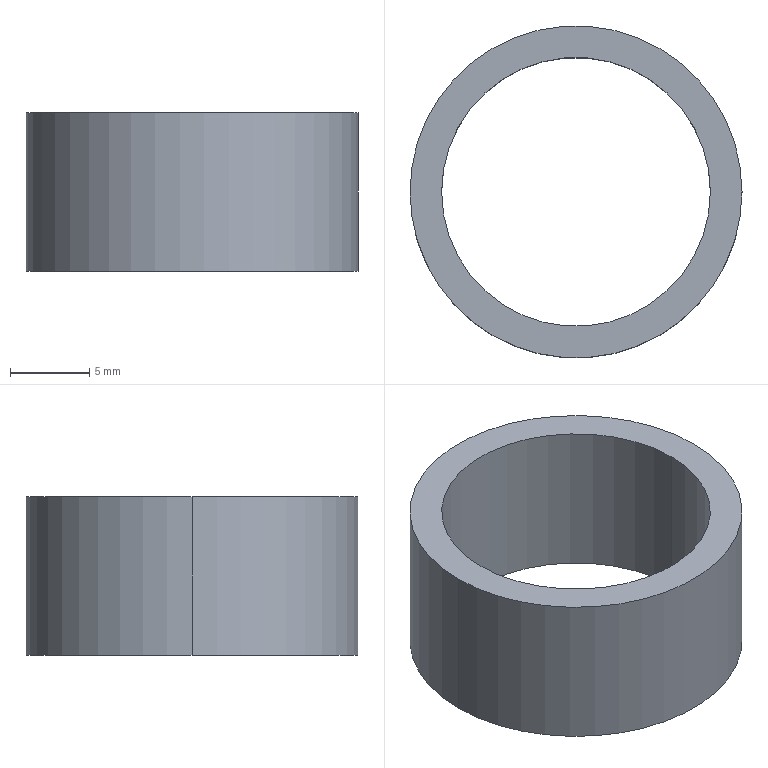Component | SolidWorks | ZDG0406-A03-P07-X1-1 | 1 solid | 6 faces | box 21 x 21 x 10 mm | volume 1194 mm3 | cylinder 4 | plane 2 | commonest cylinder face diameters 17 x2 21 x2 | material 45#
build123d program:
from build123d import *

# Parameters (mm, degrees)
SKETCH1_R           = 10.5
SKETCH1_R_2         = 8.5
BOSS_EXTRUDE1_DEPTH = 10


with BuildPart() as part:
    # Sketch1 → Boss-Extrude1 (new body)
    with BuildSketch(Plane.XY):
        Circle(SKETCH1_R)
        Circle(SKETCH1_R_2, mode=Mode.SUBTRACT)
    extrude(amount=BOSS_EXTRUDE1_DEPTH)


solid = part.part

# Placed as in the assembly
solid = solid.moved(Location((-22.5, 0, -5), (0, 0, 0)))
STEP:
#1=COLOUR_RGB('',0.7922,0.8196,0.9333);
#2=FILL_AREA_STYLE_COLOUR('',#1);
#3=FILL_AREA_STYLE('',(#2));
#4=SURFACE_STYLE_FILL_AREA(#3);
#5=SURFACE_SIDE_STYLE('',(#4));
#6=SURFACE_STYLE_USAGE(.BOTH.,#5);
#7=PRESENTATION_STYLE_ASSIGNMENT((#6));
#8=CARTESIAN_POINT('',(-1.22,-0.,0.1969));
#9=VERTEX_POINT('',#8);
#10=CARTESIAN_POINT('',(-0.5512,0.,0.1969));
#11=VERTEX_POINT('',#10);
#12=CARTESIAN_POINT('',(-0.8858,-0.,0.1969));
#13=DIRECTION('',(0.,0.,1.));
#14=DIRECTION('',(1.,0.,0.));
#15=AXIS2_PLACEMENT_3D('',#12,#13,#14);
#16=CIRCLE('',#15,0.3346);
#17=EDGE_CURVE('',#9,#11,#16,.T.);
#18=ORIENTED_EDGE('',*,*,#17,.T.);
#19=CARTESIAN_POINT('',(-0.5512,0.,-0.1969));
#20=VERTEX_POINT('',#19);
#21=CARTESIAN_POINT('',(-0.5512,0.,0.1969));
#22=DIRECTION('',(0.,0.,-1.));
#23=VECTOR('',#22,39.37);
#24=LINE('',#21,#23);
#25=EDGE_CURVE('',#11,#20,#24,.T.);
#26=ORIENTED_EDGE('',*,*,#25,.T.);
#27=CARTESIAN_POINT('',(-1.22,-0.,-0.1969));
#28=VERTEX_POINT('',#27);
#29=CARTESIAN_POINT('',(-0.8858,-0.,-0.1969));
#30=DIRECTION('',(0.,0.,1.));
#31=DIRECTION('',(1.,0.,0.));
#32=AXIS2_PLACEMENT_3D('',#29,#30,#31);
#33=CIRCLE('',#32,0.3346);
#34=EDGE_CURVE('',#28,#20,#33,.T.);
#35=ORIENTED_EDGE('',*,*,#34,.F.);
#36=CARTESIAN_POINT('',(-1.22,-0.,0.1969));
#37=DIRECTION('',(0.,0.,-1.));
#38=VECTOR('',#37,39.37);
#39=LINE('',#36,#38);
#40=EDGE_CURVE('',#9,#28,#39,.T.);
#41=ORIENTED_EDGE('',*,*,#40,.F.);
#42=EDGE_LOOP('',(#18,#26,#35,#41));
#43=FACE_OUTER_BOUND('',#42,.T.);
#44=CARTESIAN_POINT('',(-0.8858,-0.,0.1969));
#45=DIRECTION('',(0.,0.,-1.));
#46=DIRECTION('',(-1.,0.,0.));
#47=AXIS2_PLACEMENT_3D('',#44,#45,#46);
#48=CYLINDRICAL_SURFACE('',#47,0.3346);
#49=ADVANCED_FACE('',(#43),#48,.F.);
#50=CARTESIAN_POINT('',(-0.4724,0.,0.1969));
#51=VERTEX_POINT('',#50);
#52=CARTESIAN_POINT('',(-1.299,-0.,0.1969));
#53=VERTEX_POINT('',#52);
#54=CARTESIAN_POINT('',(-0.8858,-0.,0.1969));
#55=DIRECTION('',(0.,0.,1.));
#56=DIRECTION('',(1.,0.,0.));
#57=AXIS2_PLACEMENT_3D('',#54,#55,#56);
#58=CIRCLE('',#57,0.4134);
#59=EDGE_CURVE('',#51,#53,#58,.T.);
#60=ORIENTED_EDGE('',*,*,#59,.F.);
#61=CARTESIAN_POINT('',(-0.4724,0.,-0.1969));
#62=VERTEX_POINT('',#61);
#63=CARTESIAN_POINT('',(-0.4724,0.,0.1969));
#64=DIRECTION('',(0.,0.,-1.));
#65=VECTOR('',#64,39.37);
#66=LINE('',#63,#65);
#67=EDGE_CURVE('',#51,#62,#66,.T.);
#68=ORIENTED_EDGE('',*,*,#67,.T.);
#69=CARTESIAN_POINT('',(-1.299,-0.,-0.1969));
#70=VERTEX_POINT('',#69);
#71=CARTESIAN_POINT('',(-0.8858,-0.,-0.1969));
#72=DIRECTION('',(0.,0.,1.));
#73=DIRECTION('',(1.,0.,0.));
#74=AXIS2_PLACEMENT_3D('',#71,#72,#73);
#75=CIRCLE('',#74,0.4134);
#76=EDGE_CURVE('',#62,#70,#75,.T.);
#77=ORIENTED_EDGE('',*,*,#76,.T.);
#78=CARTESIAN_POINT('',(-1.299,-0.,0.1969));
#79=DIRECTION('',(0.,0.,-1.));
#80=VECTOR('',#79,39.37);
#81=LINE('',#78,#80);
#82=EDGE_CURVE('',#53,#70,#81,.T.);
#83=ORIENTED_EDGE('',*,*,#82,.F.);
#84=EDGE_LOOP('',(#60,#68,#77,#83));
#85=FACE_OUTER_BOUND('',#84,.T.);
#86=CARTESIAN_POINT('',(-0.8858,-0.,0.1969));
#87=DIRECTION('',(0.,0.,-1.));
#88=DIRECTION('',(-1.,0.,0.));
#89=AXIS2_PLACEMENT_3D('',#86,#87,#88);
#90=CYLINDRICAL_SURFACE('',#89,0.4134);
#91=ADVANCED_FACE('',(#85),#90,.T.);
#92=CARTESIAN_POINT('',(-0.8858,-0.,0.1969));
#93=DIRECTION('',(0.,0.,1.));
#94=DIRECTION('',(1.,0.,0.));
#95=AXIS2_PLACEMENT_3D('',#92,#93,#94);
#96=CIRCLE('',#95,0.4134);
#97=EDGE_CURVE('',#53,#51,#96,.T.);
#98=ORIENTED_EDGE('',*,*,#97,.T.);
#99=ORIENTED_EDGE('',*,*,#59,.T.);
#100=EDGE_LOOP('',(#98,#99));
#101=FACE_OUTER_BOUND('',#100,.T.);
#102=ORIENTED_EDGE('',*,*,#17,.F.);
#103=CARTESIAN_POINT('',(-0.8858,-0.,0.1969));
#104=DIRECTION('',(0.,0.,1.));
#105=DIRECTION('',(1.,0.,0.));
#106=AXIS2_PLACEMENT_3D('',#103,#104,#105);
#107=CIRCLE('',#106,0.3346);
#108=EDGE_CURVE('',#11,#9,#107,.T.);
#109=ORIENTED_EDGE('',*,*,#108,.F.);
#110=EDGE_LOOP('',(#102,#109));
#111=FACE_BOUND('',#110,.T.);
#112=CARTESIAN_POINT('',(-0.8858,-0.,0.1969));
#113=DIRECTION('',(0.,0.,1.));
#114=DIRECTION('',(1.,0.,0.));
#115=AXIS2_PLACEMENT_3D('',#112,#113,#114);
#116=PLANE('',#115);
#117=ADVANCED_FACE('',(#101,#111),#116,.T.);
#118=CARTESIAN_POINT('',(-0.8858,-0.,-0.1969));
#119=DIRECTION('',(0.,0.,1.));
#120=DIRECTION('',(1.,0.,0.));
#121=AXIS2_PLACEMENT_3D('',#118,#119,#120);
#122=CIRCLE('',#121,0.4134);
#123=EDGE_CURVE('',#70,#62,#122,.T.);
#124=ORIENTED_EDGE('',*,*,#123,.F.);
#125=ORIENTED_EDGE('',*,*,#76,.F.);
#126=EDGE_LOOP('',(#124,#125));
#127=FACE_OUTER_BOUND('',#126,.T.);
#128=ORIENTED_EDGE('',*,*,#34,.T.);
#129=CARTESIAN_POINT('',(-0.8858,-0.,-0.1969));
#130=DIRECTION('',(0.,0.,1.));
#131=DIRECTION('',(1.,0.,0.));
#132=AXIS2_PLACEMENT_3D('',#129,#130,#131);
#133=CIRCLE('',#132,0.3346);
#134=EDGE_CURVE('',#20,#28,#133,.T.);
#135=ORIENTED_EDGE('',*,*,#134,.T.);
#136=EDGE_LOOP('',(#128,#135));
#137=FACE_BOUND('',#136,.T.);
#138=CARTESIAN_POINT('',(-0.8858,-0.,-0.1969));
#139=DIRECTION('',(0.,0.,1.));
#140=DIRECTION('',(1.,0.,0.));
#141=AXIS2_PLACEMENT_3D('',#138,#139,#140);
#142=PLANE('',#141);
#143=ADVANCED_FACE('',(#127,#137),#142,.F.);
#144=ORIENTED_EDGE('',*,*,#67,.F.);
#145=ORIENTED_EDGE('',*,*,#97,.F.);
#146=ORIENTED_EDGE('',*,*,#82,.T.);
#147=ORIENTED_EDGE('',*,*,#123,.T.);
#148=EDGE_LOOP('',(#144,#145,#146,#147));
#149=FACE_OUTER_BOUND('',#148,.T.);
#150=CARTESIAN_POINT('',(-0.8858,-0.,0.1969));
#151=DIRECTION('',(0.,0.,-1.));
#152=DIRECTION('',(-1.,0.,0.));
#153=AXIS2_PLACEMENT_3D('',#150,#151,#152);
#154=CYLINDRICAL_SURFACE('',#153,0.4134);
#155=ADVANCED_FACE('',(#149),#154,.T.);
#156=ORIENTED_EDGE('',*,*,#25,.F.);
#157=ORIENTED_EDGE('',*,*,#108,.T.);
#158=ORIENTED_EDGE('',*,*,#40,.T.);
#159=ORIENTED_EDGE('',*,*,#134,.F.);
#160=EDGE_LOOP('',(#156,#157,#158,#159));
#161=FACE_OUTER_BOUND('',#160,.T.);
#162=CARTESIAN_POINT('',(-0.8858,-0.,0.1969));
#163=DIRECTION('',(0.,0.,-1.));
#164=DIRECTION('',(-1.,0.,0.));
#165=AXIS2_PLACEMENT_3D('',#162,#163,#164);
#166=CYLINDRICAL_SURFACE('',#165,0.3346);
#167=ADVANCED_FACE('',(#161),#166,.F.);
#168=CLOSED_SHELL('',(#49,#91,#117,#143,#155,#167));
#169=MANIFOLD_SOLID_BREP('',#168);
#170=STYLED_ITEM('',(#7),#169);
#171=PRESENTATION_LAYER_ASSIGNMENT('','',(#170));
#172=CARTESIAN_POINT('',(0.,0.,0.));
#173=DIRECTION('',(0.,0.,1.));
#174=DIRECTION('',(1.,0.,0.));
#175=AXIS2_PLACEMENT_3D('',#172,#173,#174);
#176=(LENGTH_UNIT()NAMED_UNIT(*)SI_UNIT($,.METRE.));
#177=LENGTH_MEASURE_WITH_UNIT(LENGTH_MEASURE(0.0254),#176);
#178=DIMENSIONAL_EXPONENTS(1.,0.,0.,0.,0.,0.,0.);
#179=(CONVERSION_BASED_UNIT('',#177)LENGTH_UNIT()NAMED_UNIT(#178));
#180=UNCERTAINTY_MEASURE_WITH_UNIT(LENGTH_MEASURE(0.00001),#179,'','');
#181=(NAMED_UNIT(*)PLANE_ANGLE_UNIT()SI_UNIT($,.RADIAN.));
#182=(NAMED_UNIT(*)SI_UNIT($,.STERADIAN.)SOLID_ANGLE_UNIT());
#183=(GEOMETRIC_REPRESENTATION_CONTEXT(3)GLOBAL_UNCERTAINTY_ASSIGNED_CONTEXT((#180))GLOBAL_UNIT_ASSIGNED_CONTEXT((#179,#181,#182))REPRESENTATION_CONTEXT('',''));
#184=ADVANCED_BREP_SHAPE_REPRESENTATION('',(#169,#175),#183);
#185=(LENGTH_UNIT()NAMED_UNIT(*)SI_UNIT($,.METRE.));
#186=LENGTH_MEASURE_WITH_UNIT(LENGTH_MEASURE(0.0254),#185);
#187=DIMENSIONAL_EXPONENTS(1.,0.,0.,0.,0.,0.,0.);
#188=(CONVERSION_BASED_UNIT('',#186)LENGTH_UNIT()NAMED_UNIT(#187));
#189=UNCERTAINTY_MEASURE_WITH_UNIT(LENGTH_MEASURE(0.00001),#188,'','');
#190=(NAMED_UNIT(*)PLANE_ANGLE_UNIT()SI_UNIT($,.RADIAN.));
#191=(NAMED_UNIT(*)SI_UNIT($,.STERADIAN.)SOLID_ANGLE_UNIT());
#192=(GEOMETRIC_REPRESENTATION_CONTEXT(3)GLOBAL_UNCERTAINTY_ASSIGNED_CONTEXT((#189))GLOBAL_UNIT_ASSIGNED_CONTEXT((#188,#190,#191))REPRESENTATION_CONTEXT('',''));
#193=MECHANICAL_DESIGN_GEOMETRIC_PRESENTATION_REPRESENTATION('',(#170),#192);